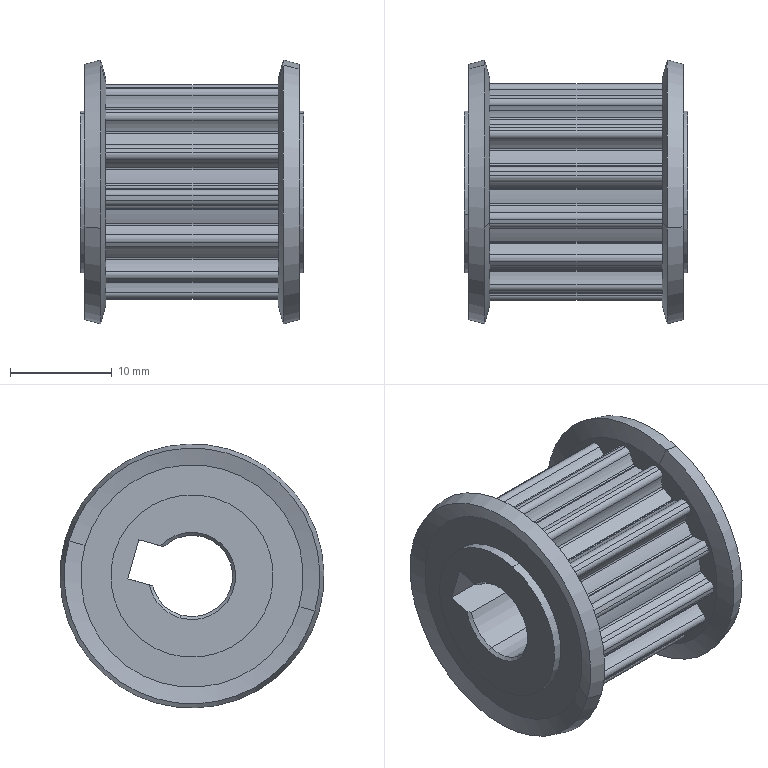Component | SolidWorks | EBJ22-S5M150-14-A-H-d8-1 | 1 solid | 159 faces | volume 5654 mm3 | cylinder 132 | cone 18 | plane 9 | commonest cylinder face diameters 1.1 x34 0.5 x32 6.55 x30 21.32 x15 17.78 x14 16 x4 8 x3